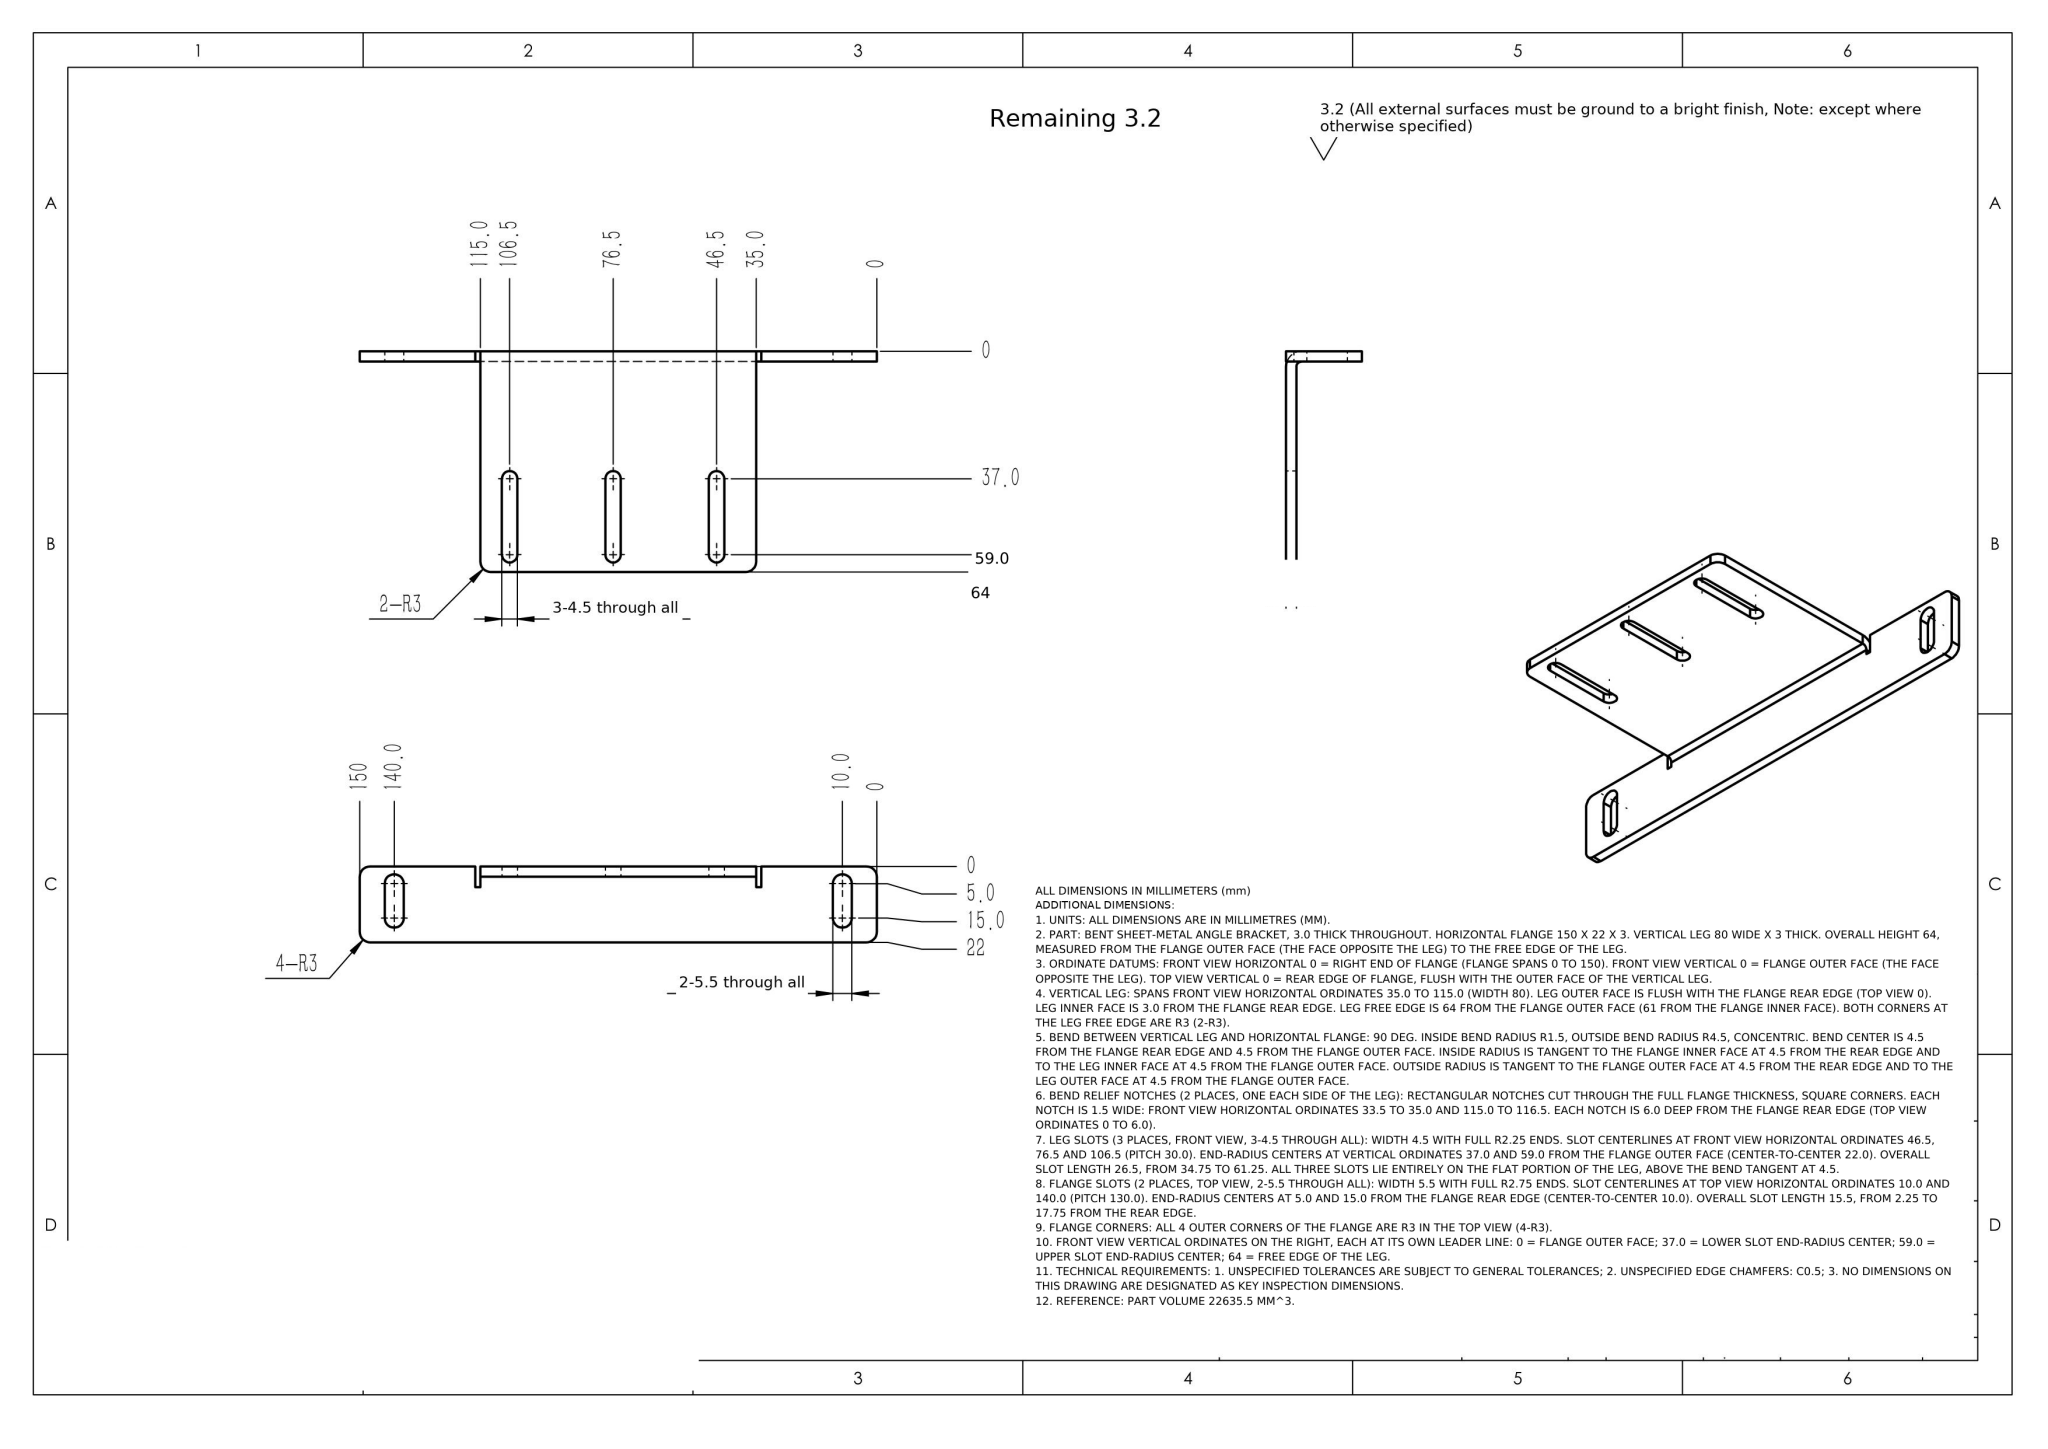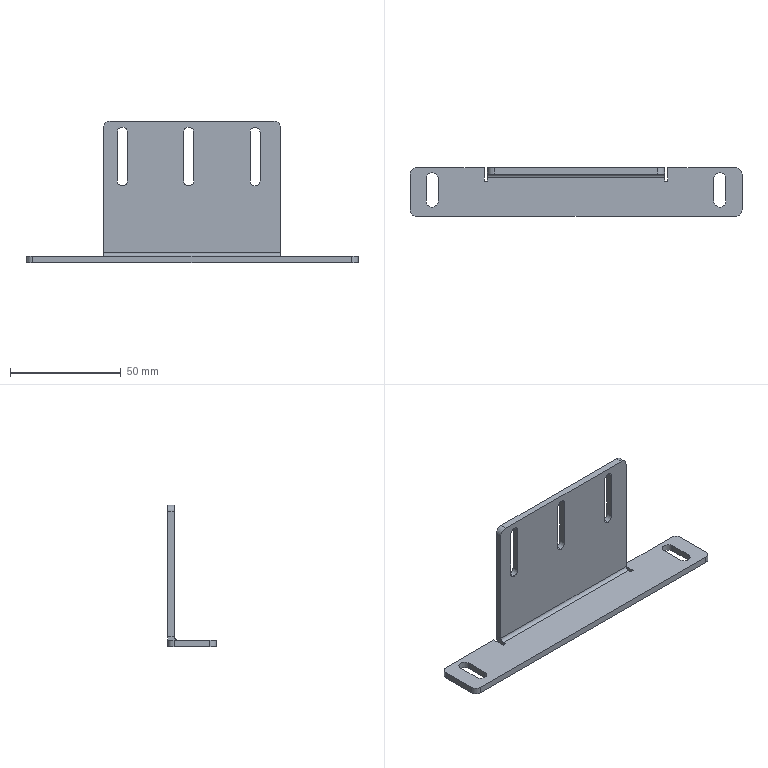Part | NX | mm | 1 solid | 51 faces | box 150 x 22 x 64 mm | volume 22636 mm3 | plane 30 | cylinder 21 | commonest cylinder face diameters 4.5 x9 6 x6 5.5 x4 9 x1 3 x1